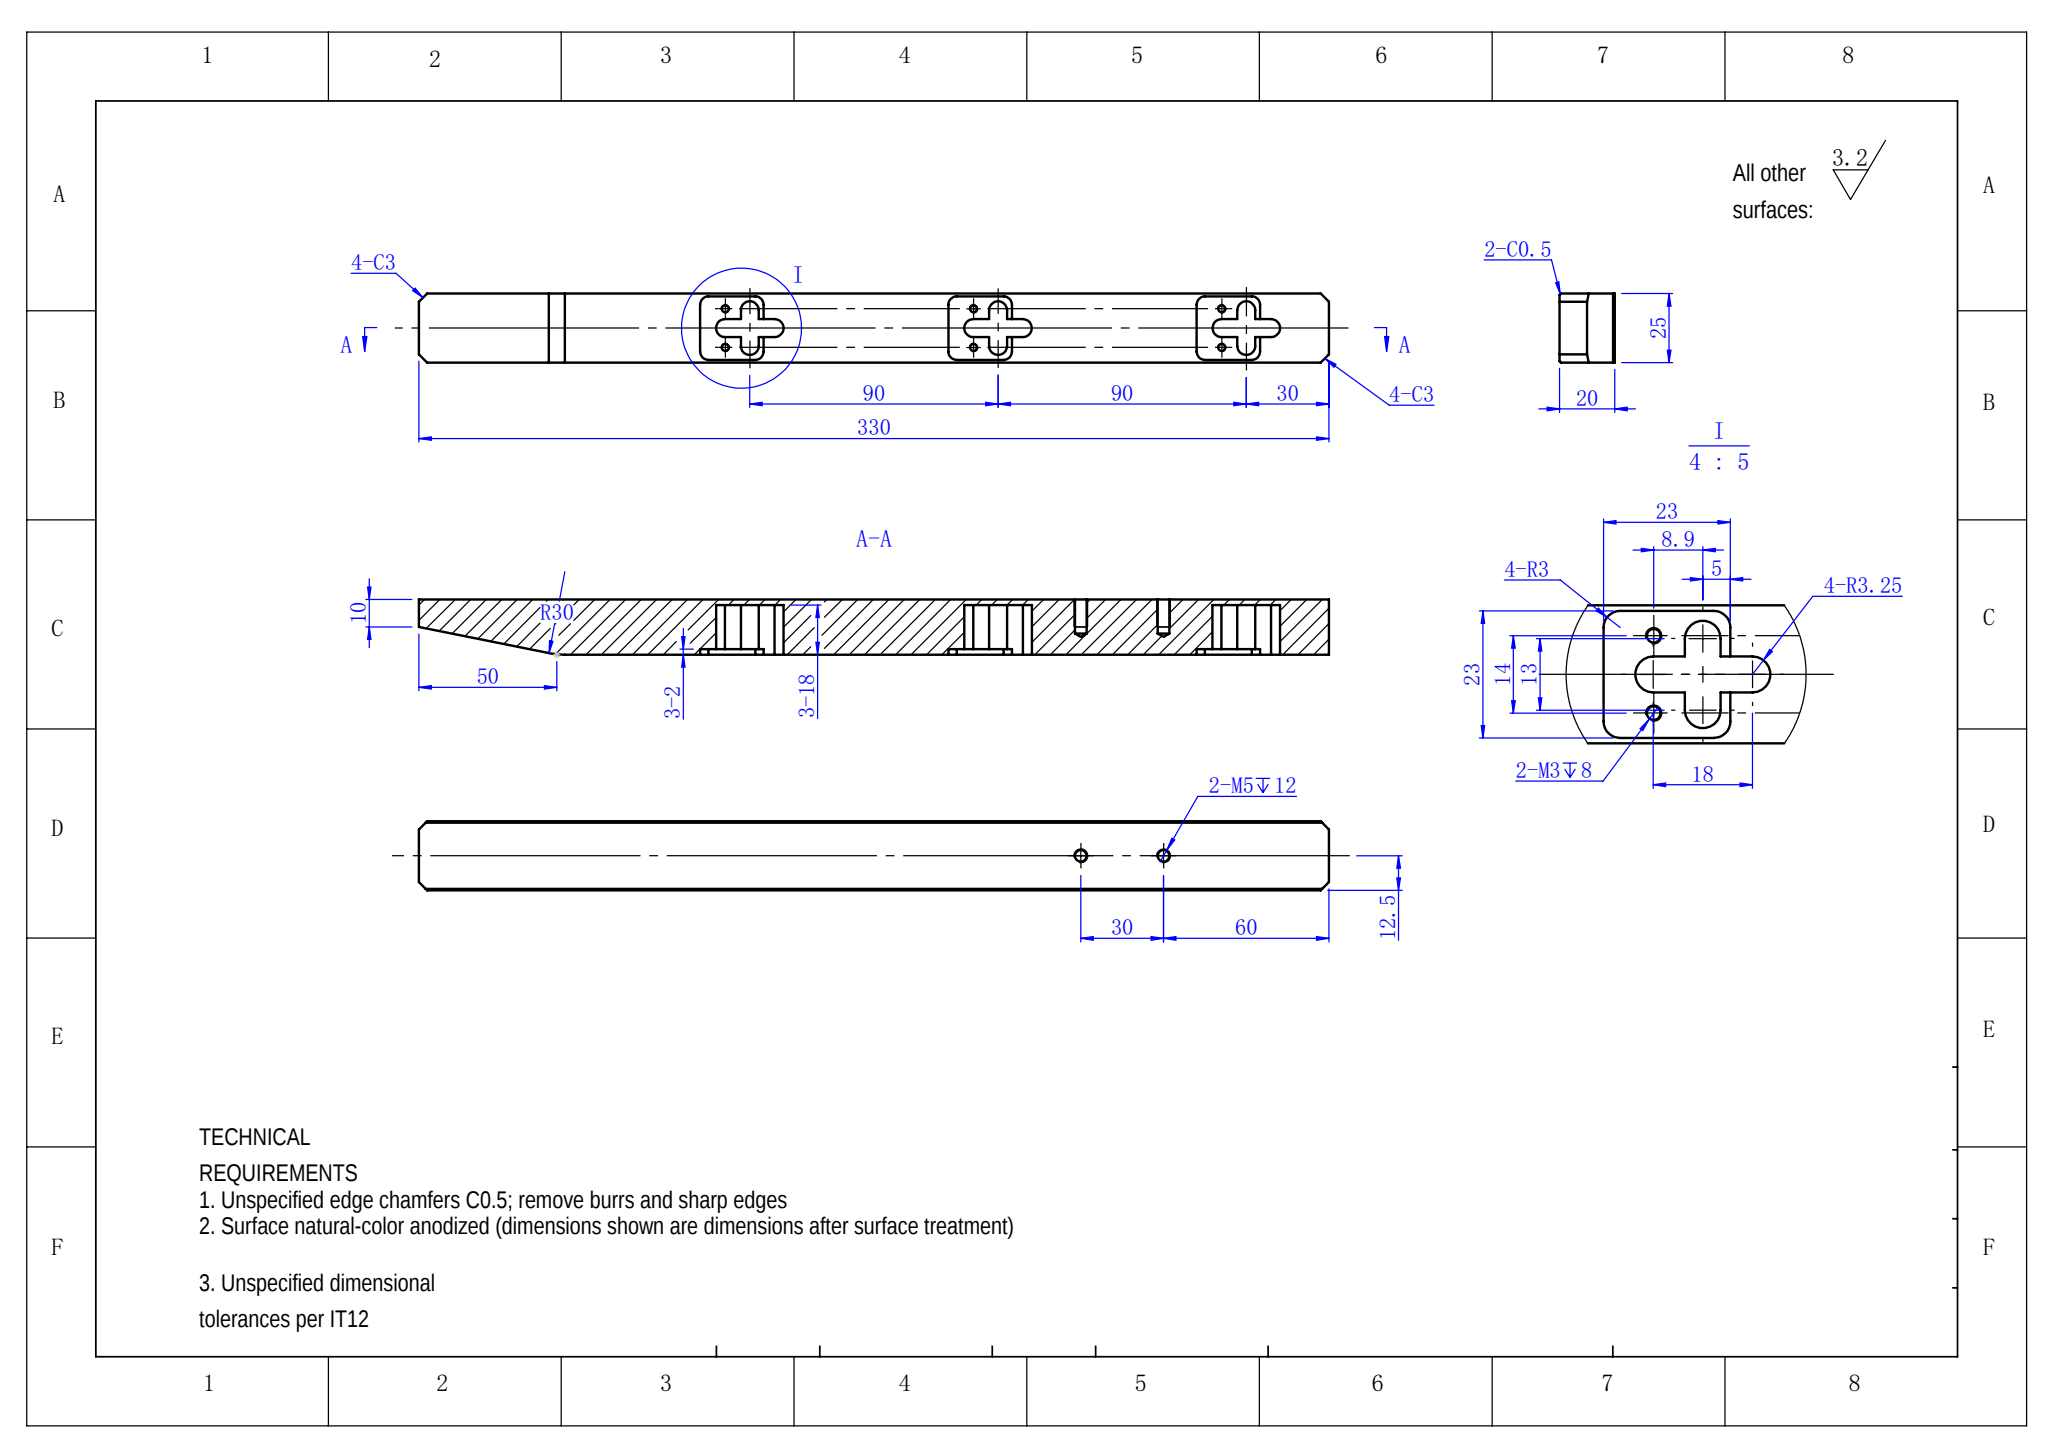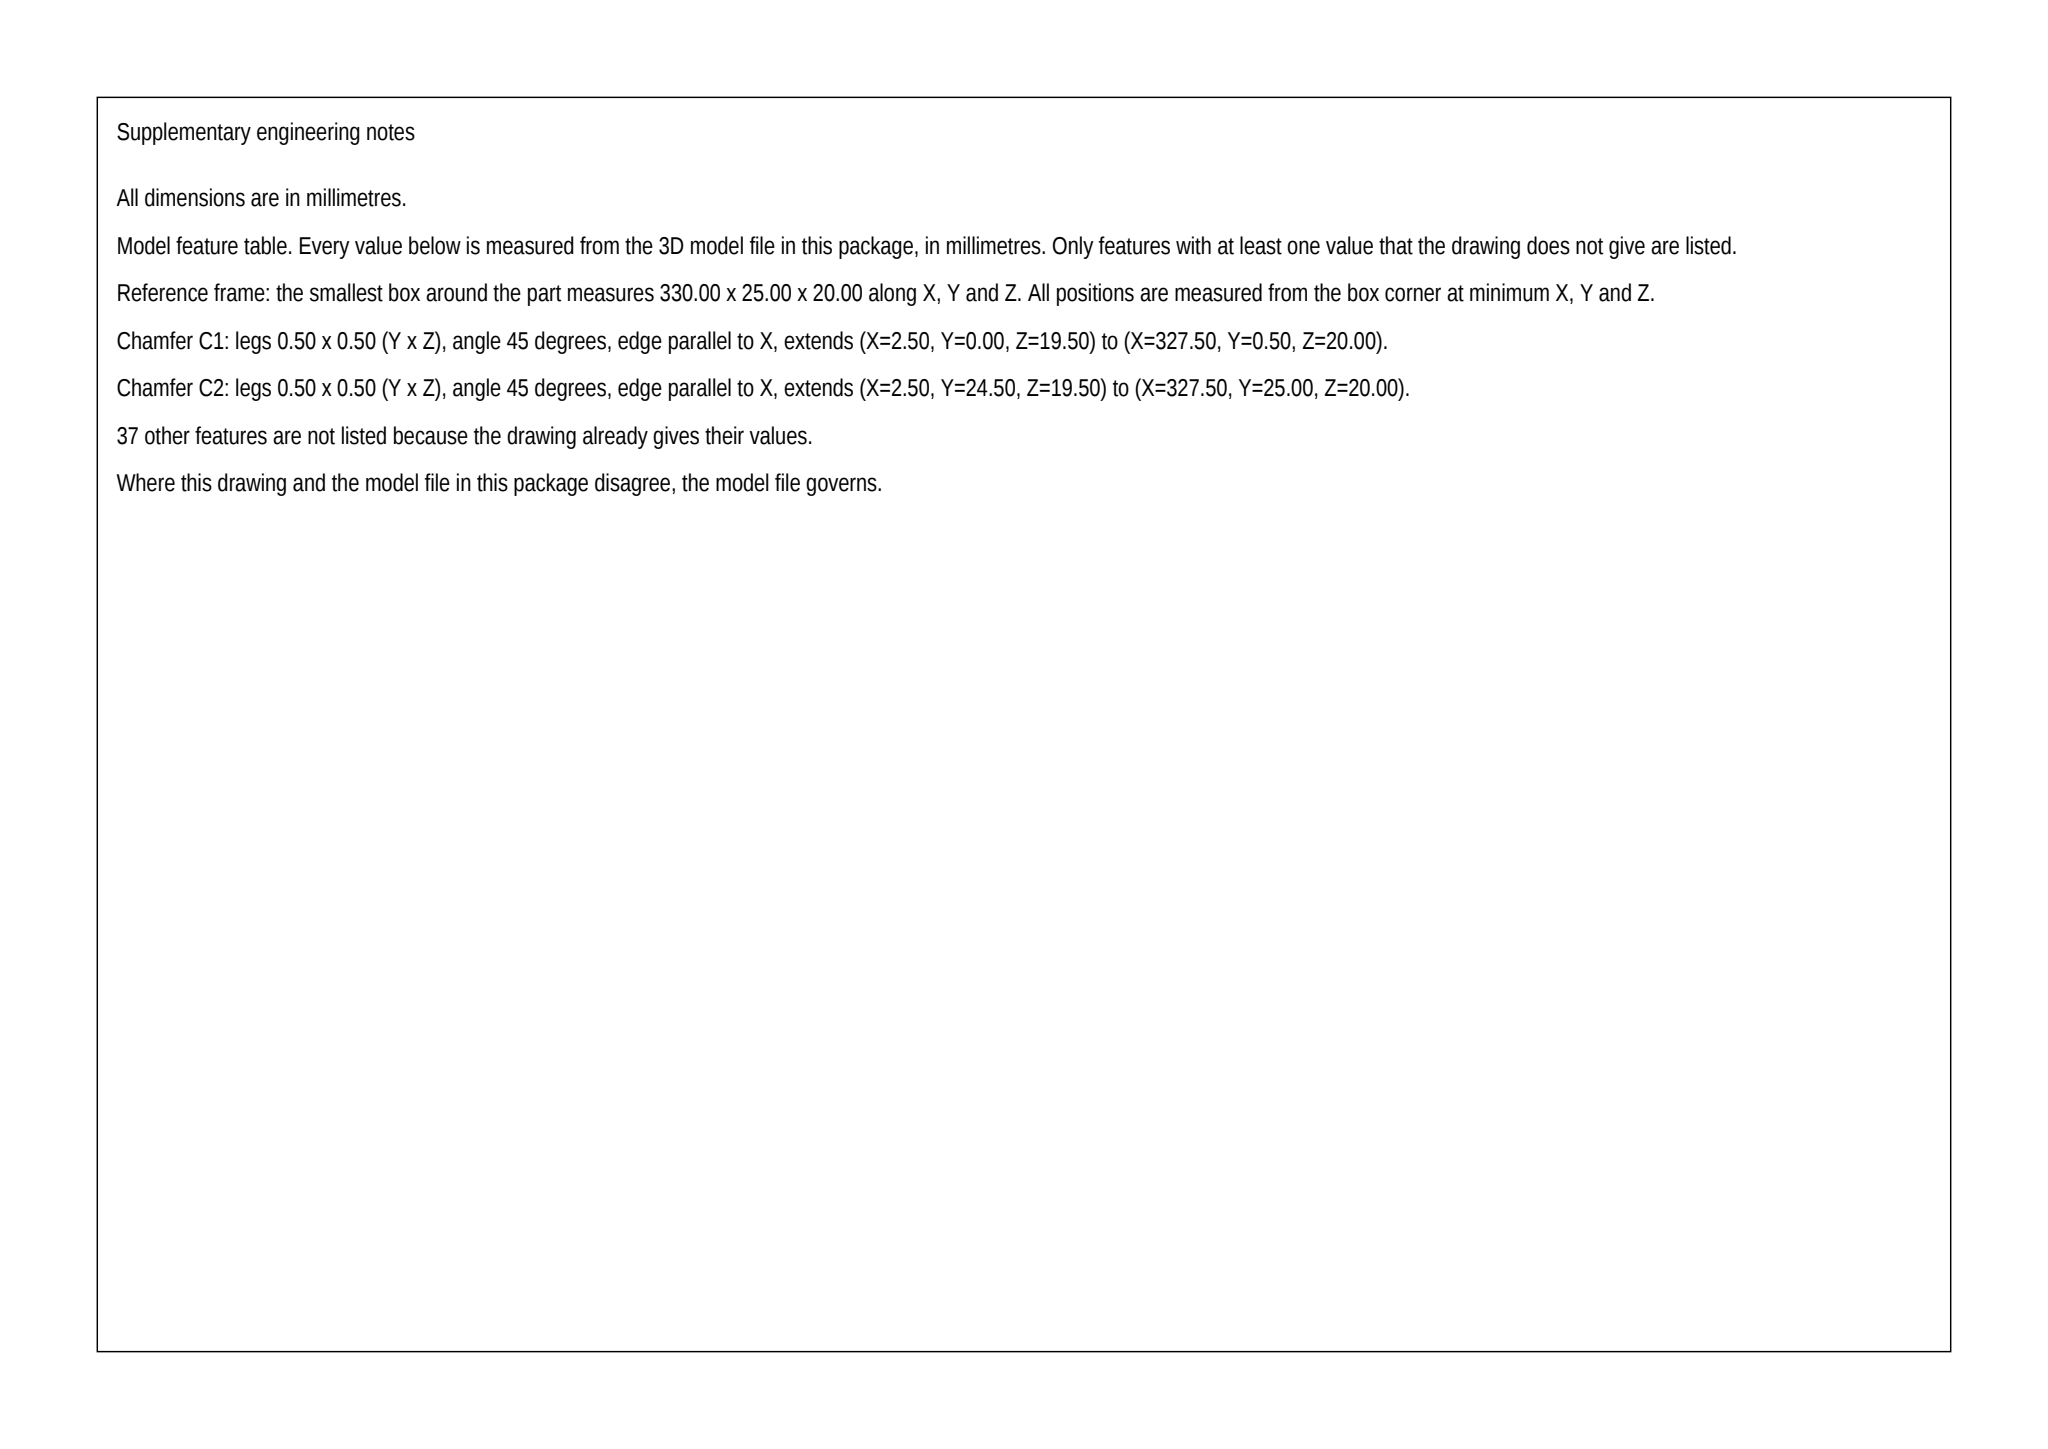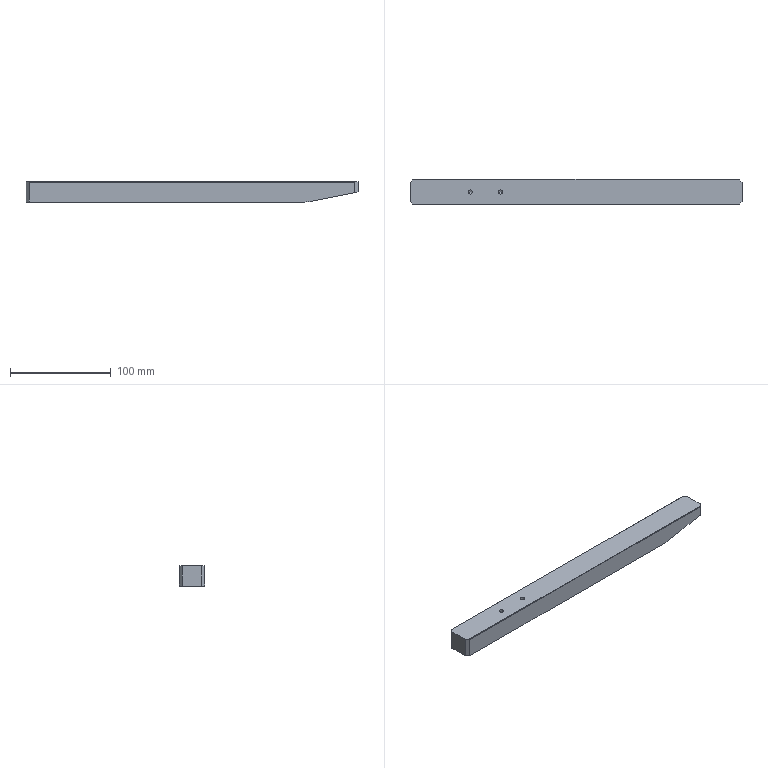Part | SolidWorks | mm | 1 solid | 118 faces | box 330 x 25 x 20 mm | volume 143594 mm3 | plane 58 | cylinder 44 | cone 16 | commonest cylinder face diameters 6.5 x15 2.5 x12 6 x12 4.2 x4 60 x1
build123d program:
from build123d import *

# Parameters (mm, degrees)
SKETCH1_W                  = 330
SKETCH1_H                  = 25
BOSS_EXTRUDE1_DEPTH        = 20
CUT_EXTRUDE1_DEPTH         = 18
CUT_EXTRUDE2_DEPTH         = 18
CUT_EXTRUDE3_DEPTH         = 2
M3_TAPPED_HOLE1_AT_2_COUNT = 2
M3_TAPPED_HOLE1_AT_2_PITCH = 14
LPATTERN1_COUNT            = 3
LPATTERN1_PITCH            = 90
M5_TAPPED_HOLE1_D          = 4.2
M5_TAPPED_HOLE1_DEPTH      = 12.4
M5_TAPPED_HOLE1_TIP        = 1.262
CHAMFER1_SIZE              = 50
CHAMFER1_SIZE2             = 10
FILLET1_R                  = 30
CHAMFER2_SIZE              = 0.5
CHAMFER3_SIZE              = 3


with BuildPart() as part:
    # Sketch1 → Boss-Extrude1 (new body)
    with BuildSketch(Plane.XY):
        with Locations((165, 0)):
            Rectangle(SKETCH1_W, SKETCH1_H)
    extrude(amount=BOSS_EXTRUDE1_DEPTH)

    # Sketch2 → Cut-Extrude1 (cut)
    with BuildSketch(Plane(origin=(0, 0, 0), x_dir=(-1, 0, 0), z_dir=(0, 0, -1))):
        with BuildLine():
            Line((-39, 3.25), (-21, 3.25))
            ThreePointArc((-21, 3.25), (-17.75, 0), (-21, -3.25))
            Line((-21, -3.25), (-39, -3.25))
            ThreePointArc((-39, -3.25), (-42.25, 0), (-39, 3.25))
        make_face()
    cut_extrude1 = extrude(amount=-CUT_EXTRUDE1_DEPTH, mode=Mode.SUBTRACT)

    # Sketch3 → Cut-Extrude2 (cut)
    with BuildSketch(Plane(origin=(0, 0, 0), x_dir=(-1, 0, 0), z_dir=(0, 0, -1))):
        with BuildLine():
            Line((-33.25, -6.5), (-33.25, 6.5))
            ThreePointArc((-33.25, 6.5), (-30, 9.75), (-26.75, 6.5))
            Line((-26.75, 6.5), (-26.75, -6.5))
            ThreePointArc((-26.75, -6.5), (-30, -9.75), (-33.25, -6.5))
        make_face()
    cut_extrude2 = extrude(amount=-CUT_EXTRUDE2_DEPTH, mode=Mode.SUBTRACT)

    # Sketch4 → Cut-Extrude3 (cut)
    with BuildSketch(Plane(origin=(0, 0, 0), x_dir=(-1, 0, 0), z_dir=(0, 0, -1))):
        with BuildLine():
            Line((-28, 11.5), (-45, 11.5))
            ThreePointArc((-45, 11.5), (-47.121, 10.621), (-48, 8.5))
            Line((-48, 8.5), (-48, -8.5))
            ThreePointArc((-48, -8.5), (-47.121, -10.621), (-45, -11.5))
            Line((-45, -11.5), (-28, -11.5))
            ThreePointArc((-28, -11.5), (-25.879, -10.621), (-25, -8.5))
            Line((-25, -8.5), (-25, 8.5))
            ThreePointArc((-25, 8.5), (-25.879, 10.621), (-28, 11.5))
        make_face()
    cut_extrude3 = extrude(amount=-CUT_EXTRUDE3_DEPTH, mode=Mode.SUBTRACT)

    # Sketch6 → M3 Tapped Hole1 (revolve, cut)
    with BuildSketch(Plane(origin=(38.9, -7, 2), x_dir=(0, 1, 0), z_dir=(1, 0, 0))):
        Polygon((0, 0), (0, 8.251), (1.25, 7.5), (1.25, 0), align=None)
    m3_tapped_hole1 = revolve(axis=Axis((38.9, -7, -4.35), (0, 0, 1)), mode=Mode.SUBTRACT)

    # M3 Tapped Hole1 at 2: M3 Tapped Hole1 ×2
    with Locations(*[(0, i * M3_TAPPED_HOLE1_AT_2_PITCH, 0) for i in range(1, M3_TAPPED_HOLE1_AT_2_COUNT)]):
        add(m3_tapped_hole1, mode=Mode.SUBTRACT)

    # LPattern1: Cut-Extrude1, Cut-Extrude2, Cut-Extrude3, M3 Tapped Hole1 ×3
    with Locations(*[(i * LPATTERN1_PITCH, 0, 0) for i in range(1, LPATTERN1_COUNT)]):
        add(cut_extrude1, mode=Mode.SUBTRACT)
        add(cut_extrude2, mode=Mode.SUBTRACT)
        add(cut_extrude3, mode=Mode.SUBTRACT)
        add(m3_tapped_hole1, mode=Mode.SUBTRACT)

    # LPattern1 copy 1 sketch → LPattern1 copy 1 (revolve, cut)
    with BuildSketch(Plane(origin=(128.9, 7, 2), x_dir=(0, 1, 0), z_dir=(1, 0, 0))):
        Polygon((0, 0), (0, 8.251), (1.25, 7.5), (1.25, 0), align=None)
    revolve(axis=Axis((128.9, 7, -4.35), (0, 0, 1)), mode=Mode.SUBTRACT)

    # LPattern1 copy 2 sketch → LPattern1 copy 2 (revolve, cut)
    with BuildSketch(Plane(origin=(218.9, 7, 2), x_dir=(0, 1, 0), z_dir=(1, 0, 0))):
        Polygon((0, 0), (0, 8.251), (1.25, 7.5), (1.25, 0), align=None)
    revolve(axis=Axis((218.9, 7, -4.35), (0, 0, 1)), mode=Mode.SUBTRACT)

    # M5 Tapped Hole1
    with Locations(Plane.XY.offset(20)):
        with Locations((60, 0), (90, 0)):
            Hole(M5_TAPPED_HOLE1_D / 2, depth=M5_TAPPED_HOLE1_DEPTH)
            with Locations((0, 0, -(M5_TAPPED_HOLE1_DEPTH + M5_TAPPED_HOLE1_TIP / 2))):  # 118° drill point
                Cone(0, M5_TAPPED_HOLE1_D / 2, M5_TAPPED_HOLE1_TIP, mode=Mode.SUBTRACT)

    # Chamfer1
    chamfer1_edges = [part.edges().sort_by_distance(p)[0] for p in [
        (330, 0, 0),
    ]]
    chamfer1_side = [part.faces().sort_by_distance(p)[0] for p in [
        (175.219, 0, 0),
    ]]
    chamfer(chamfer1_edges, length=CHAMFER1_SIZE, length2=CHAMFER1_SIZE2, reference=chamfer1_side[0])

    # Fillet1
    fillet1_edges = [part.edges().sort_by_distance(p)[0] for p in [
        (280, 0, 0),
    ]]
    fillet(fillet1_edges, radius=FILLET1_R)

    # Chamfer2
    chamfer2_edges = [part.edges().sort_by_distance(p)[0] for p in [
        (165, 12.5, 20),
        (165, -12.5, 20),
    ]]
    chamfer(chamfer2_edges, length=CHAMFER2_SIZE)

    # Chamfer3
    chamfer3_edges = [part.edges().sort_by_distance(p)[0] for p in [
        (330, -12.5, 14.75),
        (330, 12.5, 14.75),
        (0, -12.5, 9.75),
        (0, 12.5, 9.75),
    ]]
    chamfer(chamfer3_edges, length=CHAMFER3_SIZE)


solid = part.part